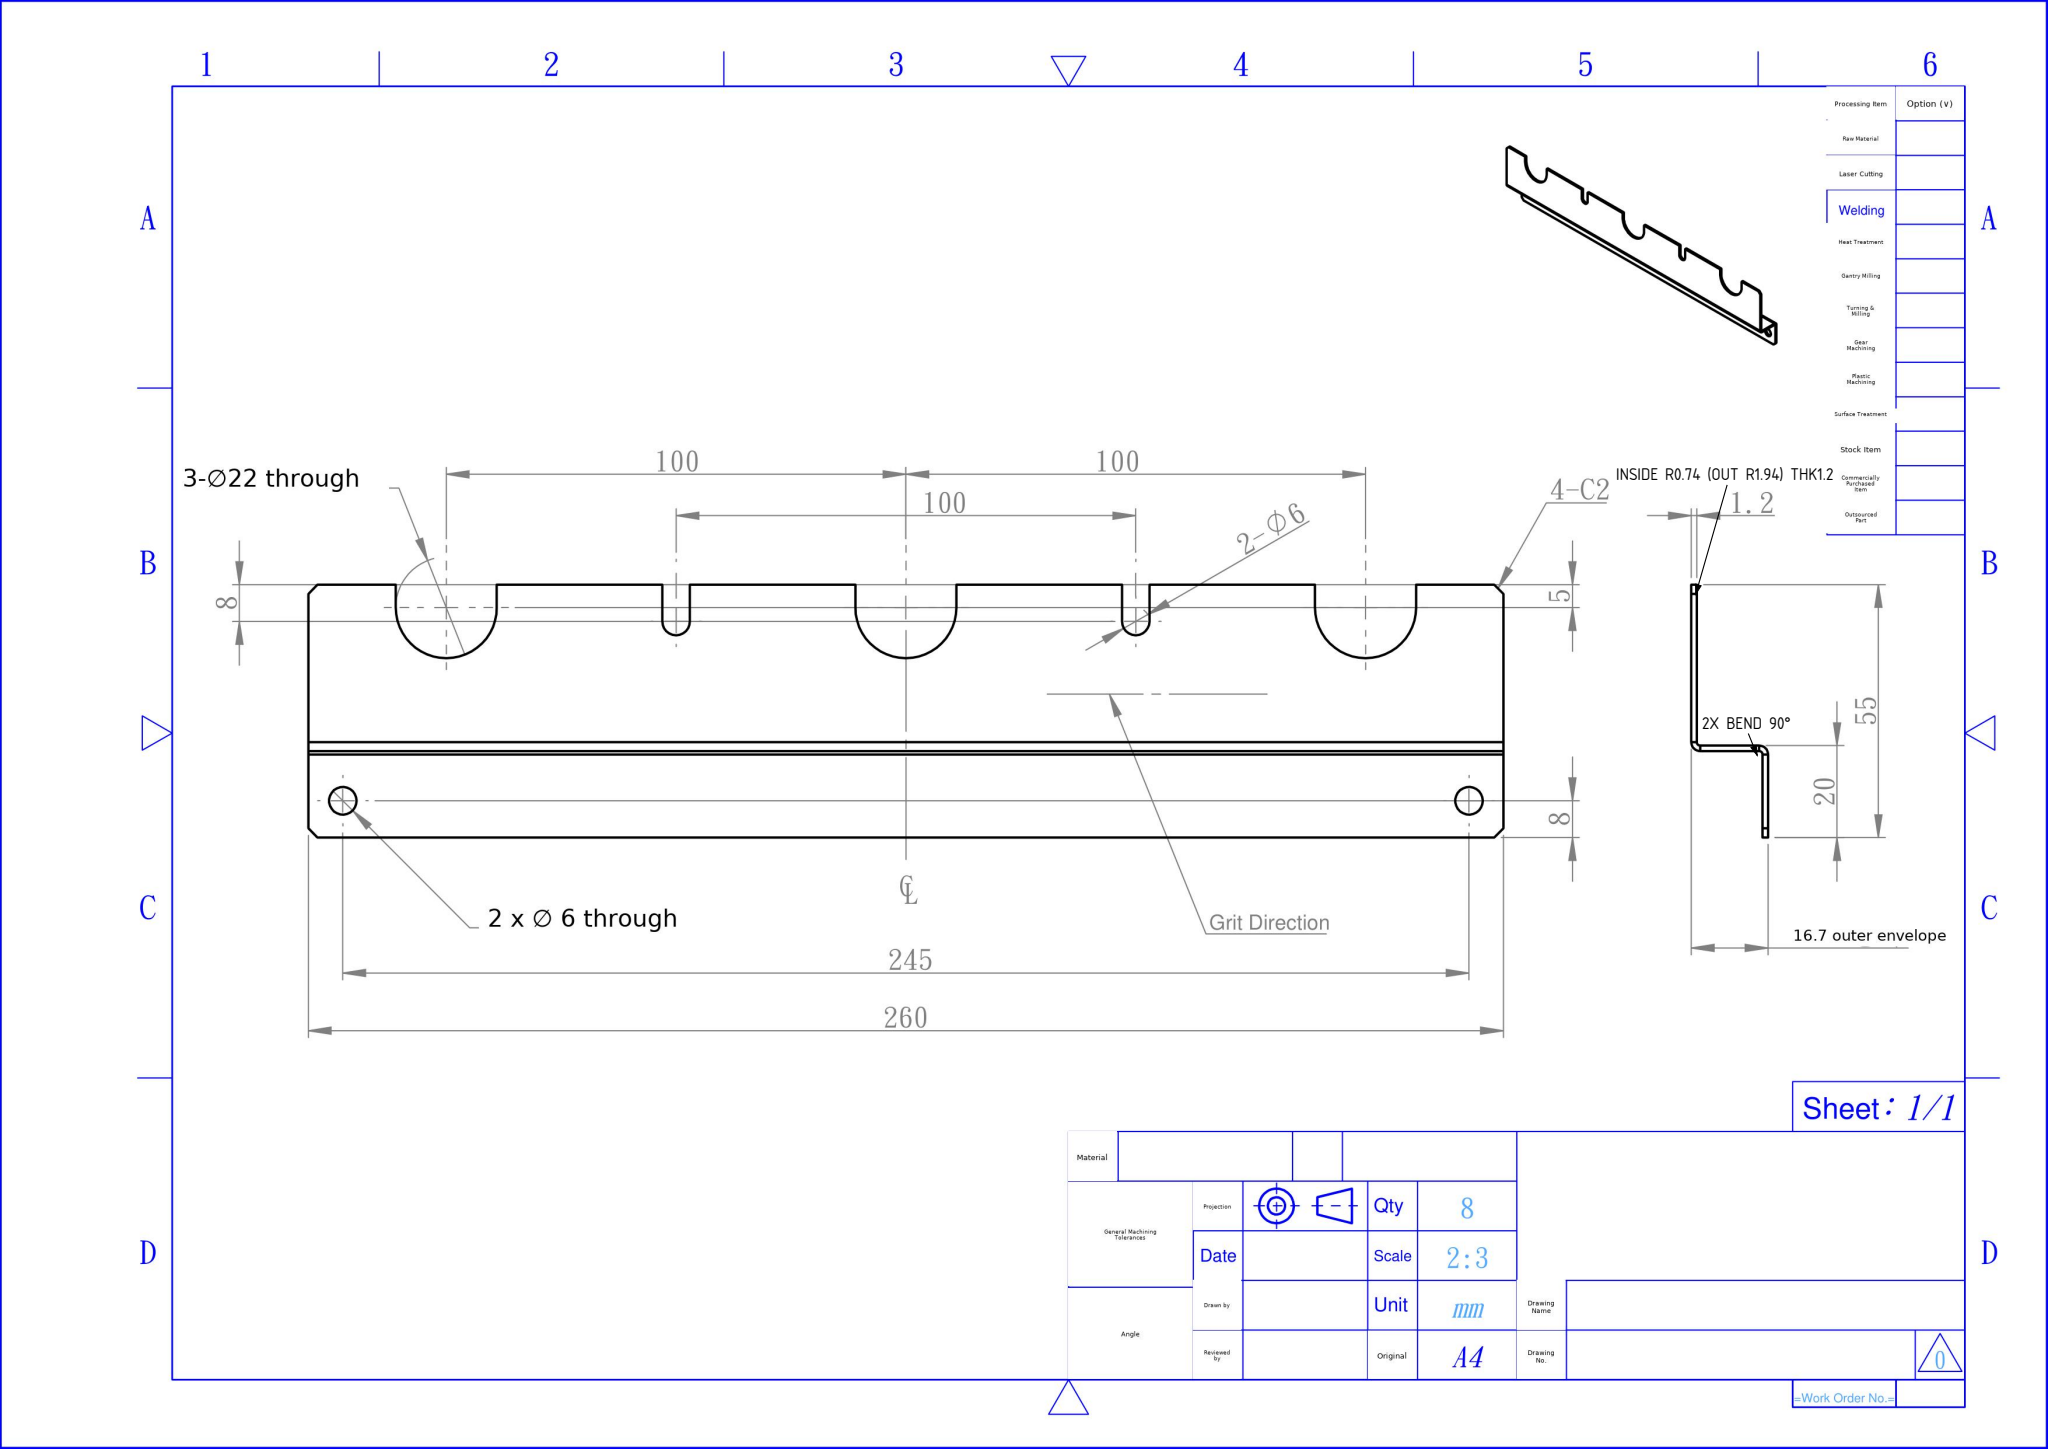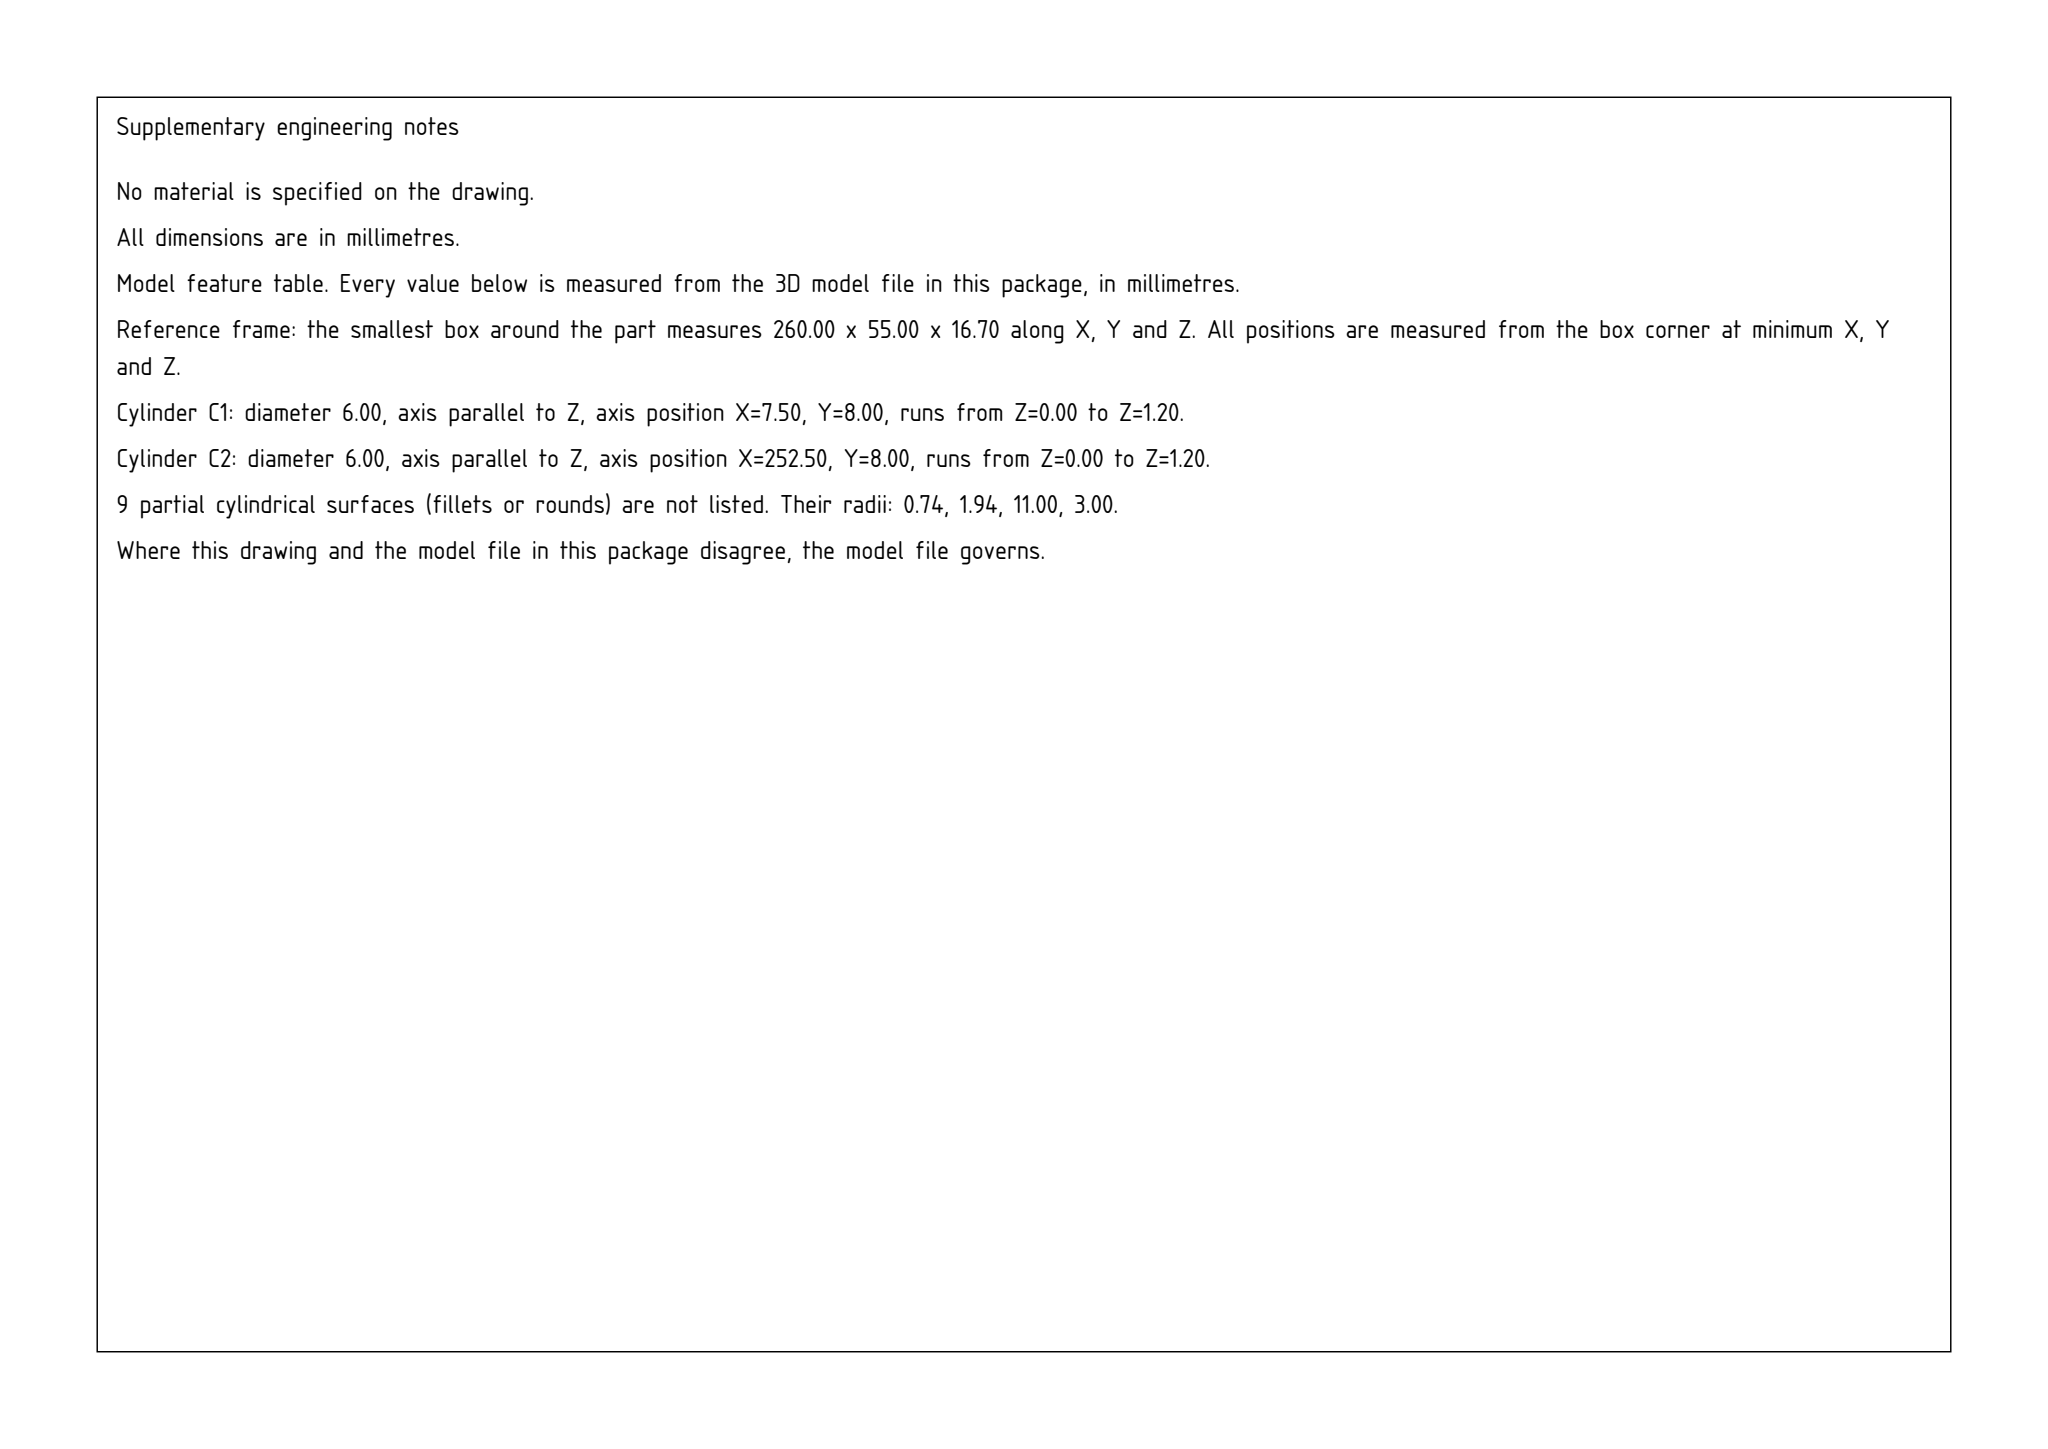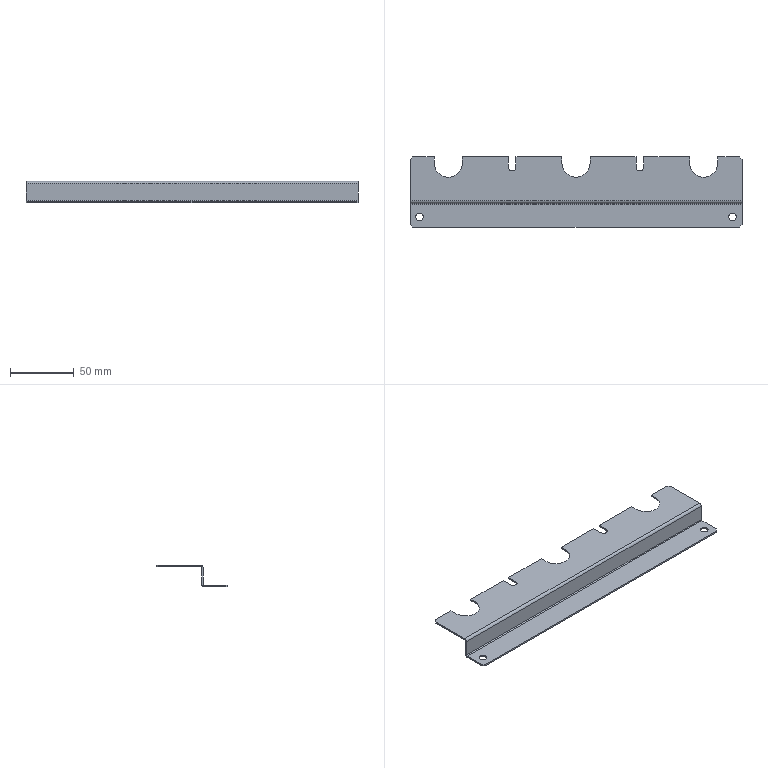Part | SolidWorks | mm | 1 solid | 50 faces | box 260 x 55 x 16.7 mm | volume 20331 mm3 | plane 37 | cylinder 13 | commonest cylinder face diameters 6 x6 22 x3 3.873 x2 1.473 x2
Drawing notes:
ALL BENDS: INSIDE R0.74 (OUTSIDE R1.94), MATL THK 1.2 | from the solid: cylinders dia 1.473 (R0.737) and dia 3.873 (R1.937) along x at bend lines y18.06/z1.94 and y20.74/z14.76; thk = z planes 0 to 1.2
BOTH FORM BENDS 90° - SEE SIDE VIEW | from the solid: faces z=0/1.2 and z=15.5/16.7 normal to z, y=18.8/20.0 normal to y: flanges mutually perpendicular